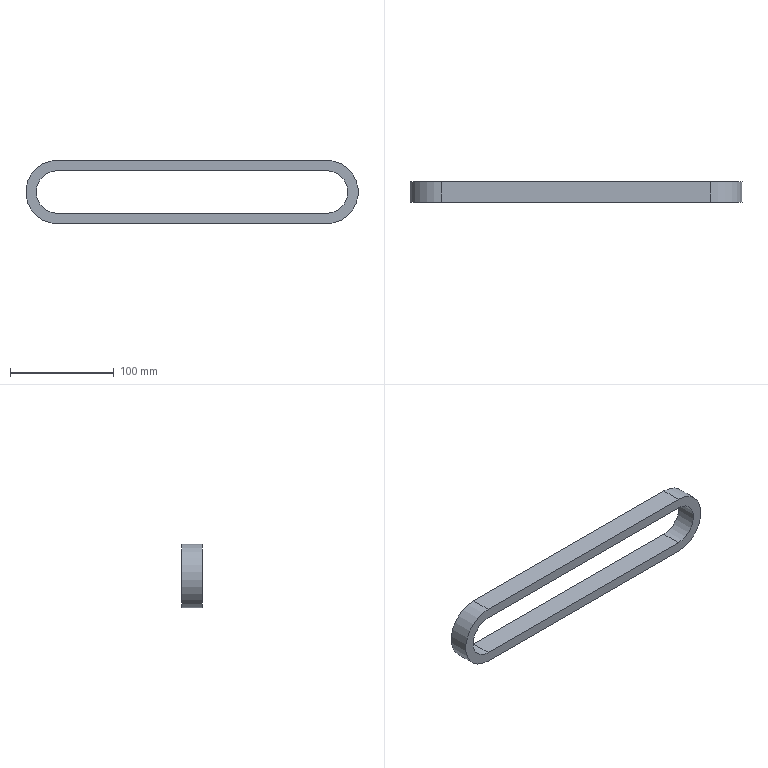Component | NX | MODEL3 | 1 solid | 10 faces | box 320 x 20 x 61 mm | volume 135644 mm3 | plane 6 | cylinder 4 | commonest cylinder face diameters 41 x2 61 x2
STEP:
#1=CARTESIAN_POINT('',(0.,0.,0.));
#2=DIRECTION('',(0.,0.,1.));
#3=DIRECTION('',(1.,0.,0.));
#4=AXIS2_PLACEMENT_3D('',#1,#2,#3);
#5=CARTESIAN_POINT('',(989.5,-5.069,-212.891));
#6=VERTEX_POINT('',#5);
#7=CARTESIAN_POINT('',(730.5,-5.069,-212.891));
#8=VERTEX_POINT('',#7);
#9=CARTESIAN_POINT('',(989.5,-5.069,-212.891));
#10=DIRECTION('',(-1.,0.,0.));
#11=VECTOR('',#10,1.);
#12=LINE('',#9,#11);
#13=CARTESIAN_POINT('',(989.5,-25.069,-212.891));
#14=DIRECTION('',(-0.,0.,-1.));
#15=DIRECTION('',(1.,0.,-0.));
#16=AXIS2_PLACEMENT_3D('',#13,#14,#15);
#17=PLANE('',#16);
#18=CARTESIAN_POINT('',(0.,-20.));
#19=DIRECTION('',(-1.,0.));
#20=VECTOR('',#19,1.);
#21=LINE('',#18,#20);
#22=(GEOMETRIC_REPRESENTATION_CONTEXT(2)PARAMETRIC_REPRESENTATION_CONTEXT()REPRESENTATION_CONTEXT('',''));
#23=DEFINITIONAL_REPRESENTATION('',(#21),#22);
#24=PCURVE('',#17,#23);
#25=CARTESIAN_POINT('',(730.5,-5.069,-192.391));
#26=DIRECTION('',(0.,1.,0.));
#27=DIRECTION('',(0.,0.,-1.));
#28=AXIS2_PLACEMENT_3D('',#25,#26,#27);
#29=PLANE('',#28);
#30=CARTESIAN_POINT('',(20.5,-259.));
#31=DIRECTION('',(-0.,1.));
#32=VECTOR('',#31,1.);
#33=LINE('',#30,#32);
#34=(GEOMETRIC_REPRESENTATION_CONTEXT(2)PARAMETRIC_REPRESENTATION_CONTEXT()REPRESENTATION_CONTEXT('',''));
#35=DEFINITIONAL_REPRESENTATION('',(#33),#34);
#36=PCURVE('',#29,#35);
#37=SURFACE_CURVE('',#12,(#24,#36),.PCURVE_S1.);
#38=EDGE_CURVE('',#6,#8,#37,.T.);
#39=ORIENTED_EDGE('',*,*,#38,.T.);
#40=CARTESIAN_POINT('',(730.5,-25.069,-212.891));
#41=VERTEX_POINT('',#40);
#42=CARTESIAN_POINT('',(730.5,-25.069,-212.891));
#43=DIRECTION('',(0.,1.,0.));
#44=VECTOR('',#43,1.);
#45=LINE('',#42,#44);
#46=CARTESIAN_POINT('',(-259.,0.));
#47=DIRECTION('',(0.,-1.));
#48=VECTOR('',#47,1.);
#49=LINE('',#46,#48);
#50=(GEOMETRIC_REPRESENTATION_CONTEXT(2)PARAMETRIC_REPRESENTATION_CONTEXT()REPRESENTATION_CONTEXT('',''));
#51=DEFINITIONAL_REPRESENTATION('',(#49),#50);
#52=PCURVE('',#17,#51);
#53=CARTESIAN_POINT('',(730.5,-25.069,-192.391));
#54=DIRECTION('',(0.,1.,0.));
#55=DIRECTION('',(0.,0.,-1.));
#56=AXIS2_PLACEMENT_3D('',#53,#54,#55);
#57=CYLINDRICAL_SURFACE('',#56,20.5);
#58=CARTESIAN_POINT('',(0.,0.));
#59=DIRECTION('',(0.,1.));
#60=VECTOR('',#59,1.);
#61=LINE('',#58,#60);
#62=(GEOMETRIC_REPRESENTATION_CONTEXT(2)PARAMETRIC_REPRESENTATION_CONTEXT()REPRESENTATION_CONTEXT('',''));
#63=DEFINITIONAL_REPRESENTATION('',(#61),#62);
#64=PCURVE('',#57,#63);
#65=SURFACE_CURVE('',#45,(#52,#64),.PCURVE_S1.);
#66=EDGE_CURVE('',#41,#8,#65,.T.);
#67=ORIENTED_EDGE('',*,*,#66,.F.);
#68=CARTESIAN_POINT('',(989.5,-25.069,-212.891));
#69=VERTEX_POINT('',#68);
#70=CARTESIAN_POINT('',(989.5,-25.069,-212.891));
#71=DIRECTION('',(-1.,0.,0.));
#72=VECTOR('',#71,1.);
#73=LINE('',#70,#72);
#74=CARTESIAN_POINT('',(0.,0.));
#75=DIRECTION('',(-1.,0.));
#76=VECTOR('',#75,1.);
#77=LINE('',#74,#76);
#78=(GEOMETRIC_REPRESENTATION_CONTEXT(2)PARAMETRIC_REPRESENTATION_CONTEXT()REPRESENTATION_CONTEXT('',''));
#79=DEFINITIONAL_REPRESENTATION('',(#77),#78);
#80=PCURVE('',#17,#79);
#81=CARTESIAN_POINT('',(730.5,-25.069,-192.391));
#82=DIRECTION('',(0.,1.,0.));
#83=DIRECTION('',(0.,0.,-1.));
#84=AXIS2_PLACEMENT_3D('',#81,#82,#83);
#85=PLANE('',#84);
#86=CARTESIAN_POINT('',(20.5,-259.));
#87=DIRECTION('',(-0.,1.));
#88=VECTOR('',#87,1.);
#89=LINE('',#86,#88);
#90=(GEOMETRIC_REPRESENTATION_CONTEXT(2)PARAMETRIC_REPRESENTATION_CONTEXT()REPRESENTATION_CONTEXT('',''));
#91=DEFINITIONAL_REPRESENTATION('',(#89),#90);
#92=PCURVE('',#85,#91);
#93=SURFACE_CURVE('',#73,(#80,#92),.PCURVE_S1.);
#94=EDGE_CURVE('',#69,#41,#93,.T.);
#95=ORIENTED_EDGE('',*,*,#94,.F.);
#96=CARTESIAN_POINT('',(989.5,-25.069,-212.891));
#97=DIRECTION('',(0.,1.,0.));
#98=VECTOR('',#97,1.);
#99=LINE('',#96,#98);
#100=CARTESIAN_POINT('',(0.,0.));
#101=DIRECTION('',(0.,-1.));
#102=VECTOR('',#101,1.);
#103=LINE('',#100,#102);
#104=(GEOMETRIC_REPRESENTATION_CONTEXT(2)PARAMETRIC_REPRESENTATION_CONTEXT()REPRESENTATION_CONTEXT('',''));
#105=DEFINITIONAL_REPRESENTATION('',(#103),#104);
#106=PCURVE('',#17,#105);
#107=CARTESIAN_POINT('',(989.5,-25.069,-192.391));
#108=DIRECTION('',(0.,1.,0.));
#109=DIRECTION('',(0.,0.,-1.));
#110=AXIS2_PLACEMENT_3D('',#107,#108,#109);
#111=CYLINDRICAL_SURFACE('',#110,20.5);
#112=CARTESIAN_POINT('',(6.283,0.));
#113=DIRECTION('',(0.,1.));
#114=VECTOR('',#113,1.);
#115=LINE('',#112,#114);
#116=(GEOMETRIC_REPRESENTATION_CONTEXT(2)PARAMETRIC_REPRESENTATION_CONTEXT()REPRESENTATION_CONTEXT('',''));
#117=DEFINITIONAL_REPRESENTATION('',(#115),#116);
#118=PCURVE('',#111,#117);
#119=SURFACE_CURVE('',#99,(#106,#118),.PCURVE_S1.);
#120=EDGE_CURVE('',#69,#6,#119,.T.);
#121=ORIENTED_EDGE('',*,*,#120,.T.);
#122=EDGE_LOOP('',(#39,#67,#95,#121));
#123=FACE_BOUND('',#122,.T.);
#124=ADVANCED_FACE('',(#123),#17,.F.);
#125=CARTESIAN_POINT('',(989.5,-25.069,-171.891));
#126=VERTEX_POINT('',#125);
#127=CARTESIAN_POINT('',(989.5,-5.069,-171.891));
#128=VERTEX_POINT('',#127);
#129=CARTESIAN_POINT('',(989.5,-25.069,-171.891));
#130=DIRECTION('',(0.,1.,0.));
#131=VECTOR('',#130,1.);
#132=LINE('',#129,#131);
#133=CARTESIAN_POINT('',(3.142,0.));
#134=DIRECTION('',(0.,1.));
#135=VECTOR('',#134,1.);
#136=LINE('',#133,#135);
#137=(GEOMETRIC_REPRESENTATION_CONTEXT(2)PARAMETRIC_REPRESENTATION_CONTEXT()REPRESENTATION_CONTEXT('',''));
#138=DEFINITIONAL_REPRESENTATION('',(#136),#137);
#139=PCURVE('',#111,#138);
#140=CARTESIAN_POINT('',(730.5,-25.069,-171.891));
#141=DIRECTION('',(0.,0.,1.));
#142=DIRECTION('',(-1.,0.,0.));
#143=AXIS2_PLACEMENT_3D('',#140,#141,#142);
#144=PLANE('',#143);
#145=CARTESIAN_POINT('',(-259.,0.));
#146=DIRECTION('',(0.,-1.));
#147=VECTOR('',#146,1.);
#148=LINE('',#145,#147);
#149=(GEOMETRIC_REPRESENTATION_CONTEXT(2)PARAMETRIC_REPRESENTATION_CONTEXT()REPRESENTATION_CONTEXT('',''));
#150=DEFINITIONAL_REPRESENTATION('',(#148),#149);
#151=PCURVE('',#144,#150);
#152=SURFACE_CURVE('',#132,(#139,#151),.PCURVE_S1.);
#153=EDGE_CURVE('',#126,#128,#152,.T.);
#154=ORIENTED_EDGE('',*,*,#153,.F.);
#155=CARTESIAN_POINT('',(989.5,-25.069,-192.391));
#156=DIRECTION('',(0.,1.,0.));
#157=DIRECTION('',(0.,0.,1.));
#158=AXIS2_PLACEMENT_3D('',#155,#156,#157);
#159=CIRCLE('',#158,20.5);
#160=CARTESIAN_POINT('',(3.142,0.));
#161=DIRECTION('',(1.,0.));
#162=VECTOR('',#161,1.);
#163=LINE('',#160,#162);
#164=(GEOMETRIC_REPRESENTATION_CONTEXT(2)PARAMETRIC_REPRESENTATION_CONTEXT()REPRESENTATION_CONTEXT('',''));
#165=DEFINITIONAL_REPRESENTATION('',(#163),#164);
#166=PCURVE('',#111,#165);
#167=CARTESIAN_POINT('',(0.,-259.));
#168=DIRECTION('',(-1.,0.));
#169=AXIS2_PLACEMENT_2D('',#167,#168);
#170=CIRCLE('',#169,20.5);
#171=(GEOMETRIC_REPRESENTATION_CONTEXT(2)PARAMETRIC_REPRESENTATION_CONTEXT()REPRESENTATION_CONTEXT('',''));
#172=DEFINITIONAL_REPRESENTATION('',(#170),#171);
#173=PCURVE('',#85,#172);
#174=SURFACE_CURVE('',#159,(#166,#173),.PCURVE_S1.);
#175=EDGE_CURVE('',#126,#69,#174,.T.);
#176=ORIENTED_EDGE('',*,*,#175,.T.);
#177=ORIENTED_EDGE('',*,*,#120,.T.);
#178=CARTESIAN_POINT('',(989.5,-5.069,-192.391));
#179=DIRECTION('',(0.,1.,0.));
#180=DIRECTION('',(0.,0.,1.));
#181=AXIS2_PLACEMENT_3D('',#178,#179,#180);
#182=CIRCLE('',#181,20.5);
#183=CARTESIAN_POINT('',(3.142,20.));
#184=DIRECTION('',(1.,0.));
#185=VECTOR('',#184,1.);
#186=LINE('',#183,#185);
#187=(GEOMETRIC_REPRESENTATION_CONTEXT(2)PARAMETRIC_REPRESENTATION_CONTEXT()REPRESENTATION_CONTEXT('',''));
#188=DEFINITIONAL_REPRESENTATION('',(#186),#187);
#189=PCURVE('',#111,#188);
#190=CARTESIAN_POINT('',(0.,-259.));
#191=DIRECTION('',(-1.,0.));
#192=AXIS2_PLACEMENT_2D('',#190,#191);
#193=CIRCLE('',#192,20.5);
#194=(GEOMETRIC_REPRESENTATION_CONTEXT(2)PARAMETRIC_REPRESENTATION_CONTEXT()REPRESENTATION_CONTEXT('',''));
#195=DEFINITIONAL_REPRESENTATION('',(#193),#194);
#196=PCURVE('',#29,#195);
#197=SURFACE_CURVE('',#182,(#189,#196),.PCURVE_S1.);
#198=EDGE_CURVE('',#128,#6,#197,.T.);
#199=ORIENTED_EDGE('',*,*,#198,.F.);
#200=EDGE_LOOP('',(#154,#176,#177,#199));
#201=FACE_BOUND('',#200,.F.);
#202=ADVANCED_FACE('',(#201),#111,.F.);
#203=CARTESIAN_POINT('',(730.5,-5.069,-171.891));
#204=VERTEX_POINT('',#203);
#205=CARTESIAN_POINT('',(730.5,-5.069,-171.891));
#206=DIRECTION('',(1.,0.,-0.));
#207=VECTOR('',#206,1.);
#208=LINE('',#205,#207);
#209=CARTESIAN_POINT('',(0.,-20.));
#210=DIRECTION('',(-1.,0.));
#211=VECTOR('',#210,1.);
#212=LINE('',#209,#211);
#213=(GEOMETRIC_REPRESENTATION_CONTEXT(2)PARAMETRIC_REPRESENTATION_CONTEXT()REPRESENTATION_CONTEXT('',''));
#214=DEFINITIONAL_REPRESENTATION('',(#212),#213);
#215=PCURVE('',#144,#214);
#216=CARTESIAN_POINT('',(-20.5,0.));
#217=DIRECTION('',(0.,-1.));
#218=VECTOR('',#217,1.);
#219=LINE('',#216,#218);
#220=(GEOMETRIC_REPRESENTATION_CONTEXT(2)PARAMETRIC_REPRESENTATION_CONTEXT()REPRESENTATION_CONTEXT('',''));
#221=DEFINITIONAL_REPRESENTATION('',(#219),#220);
#222=PCURVE('',#29,#221);
#223=SURFACE_CURVE('',#208,(#215,#222),.PCURVE_S1.);
#224=EDGE_CURVE('',#204,#128,#223,.T.);
#225=ORIENTED_EDGE('',*,*,#224,.T.);
#226=ORIENTED_EDGE('',*,*,#153,.F.);
#227=CARTESIAN_POINT('',(730.5,-25.069,-171.891));
#228=VERTEX_POINT('',#227);
#229=CARTESIAN_POINT('',(730.5,-25.069,-171.891));
#230=DIRECTION('',(1.,0.,-0.));
#231=VECTOR('',#230,1.);
#232=LINE('',#229,#231);
#233=CARTESIAN_POINT('',(0.,0.));
#234=DIRECTION('',(-1.,0.));
#235=VECTOR('',#234,1.);
#236=LINE('',#233,#235);
#237=(GEOMETRIC_REPRESENTATION_CONTEXT(2)PARAMETRIC_REPRESENTATION_CONTEXT()REPRESENTATION_CONTEXT('',''));
#238=DEFINITIONAL_REPRESENTATION('',(#236),#237);
#239=PCURVE('',#144,#238);
#240=CARTESIAN_POINT('',(-20.5,0.));
#241=DIRECTION('',(0.,-1.));
#242=VECTOR('',#241,1.);
#243=LINE('',#240,#242);
#244=(GEOMETRIC_REPRESENTATION_CONTEXT(2)PARAMETRIC_REPRESENTATION_CONTEXT()REPRESENTATION_CONTEXT('',''));
#245=DEFINITIONAL_REPRESENTATION('',(#243),#244);
#246=PCURVE('',#85,#245);
#247=SURFACE_CURVE('',#232,(#239,#246),.PCURVE_S1.);
#248=EDGE_CURVE('',#228,#126,#247,.T.);
#249=ORIENTED_EDGE('',*,*,#248,.F.);
#250=CARTESIAN_POINT('',(730.5,-25.069,-171.891));
#251=DIRECTION('',(0.,1.,0.));
#252=VECTOR('',#251,1.);
#253=LINE('',#250,#252);
#254=CARTESIAN_POINT('',(0.,0.));
#255=DIRECTION('',(0.,-1.));
#256=VECTOR('',#255,1.);
#257=LINE('',#254,#256);
#258=(GEOMETRIC_REPRESENTATION_CONTEXT(2)PARAMETRIC_REPRESENTATION_CONTEXT()REPRESENTATION_CONTEXT('',''));
#259=DEFINITIONAL_REPRESENTATION('',(#257),#258);
#260=PCURVE('',#144,#259);
#261=CARTESIAN_POINT('',(3.142,0.));
#262=DIRECTION('',(0.,1.));
#263=VECTOR('',#262,1.);
#264=LINE('',#261,#263);
#265=(GEOMETRIC_REPRESENTATION_CONTEXT(2)PARAMETRIC_REPRESENTATION_CONTEXT()REPRESENTATION_CONTEXT('',''));
#266=DEFINITIONAL_REPRESENTATION('',(#264),#265);
#267=PCURVE('',#57,#266);
#268=SURFACE_CURVE('',#253,(#260,#267),.PCURVE_S1.);
#269=EDGE_CURVE('',#228,#204,#268,.T.);
#270=ORIENTED_EDGE('',*,*,#269,.T.);
#271=EDGE_LOOP('',(#225,#226,#249,#270));
#272=FACE_BOUND('',#271,.T.);
#273=ADVANCED_FACE('',(#272),#144,.F.);
#274=CARTESIAN_POINT('',(989.5,-5.069,-222.891));
#275=VERTEX_POINT('',#274);
#276=CARTESIAN_POINT('',(730.5,-5.069,-222.891));
#277=VERTEX_POINT('',#276);
#278=CARTESIAN_POINT('',(989.5,-5.069,-222.891));
#279=DIRECTION('',(-1.,0.,0.));
#280=VECTOR('',#279,1.);
#281=LINE('',#278,#280);
#282=CARTESIAN_POINT('',(989.5,-25.069,-222.891));
#283=DIRECTION('',(-0.,0.,-1.));
#284=DIRECTION('',(1.,0.,-0.));
#285=AXIS2_PLACEMENT_3D('',#282,#283,#284);
#286=PLANE('',#285);
#287=CARTESIAN_POINT('',(0.,-20.));
#288=DIRECTION('',(-1.,0.));
#289=VECTOR('',#288,1.);
#290=LINE('',#287,#289);
#291=(GEOMETRIC_REPRESENTATION_CONTEXT(2)PARAMETRIC_REPRESENTATION_CONTEXT()REPRESENTATION_CONTEXT('',''));
#292=DEFINITIONAL_REPRESENTATION('',(#290),#291);
#293=PCURVE('',#286,#292);
#294=CARTESIAN_POINT('',(30.5,-259.));
#295=DIRECTION('',(-0.,1.));
#296=VECTOR('',#295,1.);
#297=LINE('',#294,#296);
#298=(GEOMETRIC_REPRESENTATION_CONTEXT(2)PARAMETRIC_REPRESENTATION_CONTEXT()REPRESENTATION_CONTEXT('',''));
#299=DEFINITIONAL_REPRESENTATION('',(#297),#298);
#300=PCURVE('',#29,#299);
#301=SURFACE_CURVE('',#281,(#293,#300),.PCURVE_S1.);
#302=EDGE_CURVE('',#275,#277,#301,.T.);
#303=ORIENTED_EDGE('',*,*,#302,.F.);
#304=CARTESIAN_POINT('',(989.5,-25.069,-222.891));
#305=VERTEX_POINT('',#304);
#306=CARTESIAN_POINT('',(989.5,-25.069,-222.891));
#307=DIRECTION('',(0.,1.,0.));
#308=VECTOR('',#307,1.);
#309=LINE('',#306,#308);
#310=CARTESIAN_POINT('',(0.,0.));
#311=DIRECTION('',(0.,-1.));
#312=VECTOR('',#311,1.);
#313=LINE('',#310,#312);
#314=(GEOMETRIC_REPRESENTATION_CONTEXT(2)PARAMETRIC_REPRESENTATION_CONTEXT()REPRESENTATION_CONTEXT('',''));
#315=DEFINITIONAL_REPRESENTATION('',(#313),#314);
#316=PCURVE('',#286,#315);
#317=CARTESIAN_POINT('',(989.5,-25.069,-192.391));
#318=DIRECTION('',(0.,1.,0.));
#319=DIRECTION('',(0.,0.,-1.));
#320=AXIS2_PLACEMENT_3D('',#317,#318,#319);
#321=CYLINDRICAL_SURFACE('',#320,30.5);
#322=CARTESIAN_POINT('',(6.283,0.));
#323=DIRECTION('',(0.,1.));
#324=VECTOR('',#323,1.);
#325=LINE('',#322,#324);
#326=(GEOMETRIC_REPRESENTATION_CONTEXT(2)PARAMETRIC_REPRESENTATION_CONTEXT()REPRESENTATION_CONTEXT('',''));
#327=DEFINITIONAL_REPRESENTATION('',(#325),#326);
#328=PCURVE('',#321,#327);
#329=SURFACE_CURVE('',#309,(#316,#328),.PCURVE_S1.);
#330=EDGE_CURVE('',#305,#275,#329,.T.);
#331=ORIENTED_EDGE('',*,*,#330,.F.);
#332=CARTESIAN_POINT('',(730.5,-25.069,-222.891));
#333=VERTEX_POINT('',#332);
#334=CARTESIAN_POINT('',(989.5,-25.069,-222.891));
#335=DIRECTION('',(-1.,0.,0.));
#336=VECTOR('',#335,1.);
#337=LINE('',#334,#336);
#338=CARTESIAN_POINT('',(0.,0.));
#339=DIRECTION('',(-1.,0.));
#340=VECTOR('',#339,1.);
#341=LINE('',#338,#340);
#342=(GEOMETRIC_REPRESENTATION_CONTEXT(2)PARAMETRIC_REPRESENTATION_CONTEXT()REPRESENTATION_CONTEXT('',''));
#343=DEFINITIONAL_REPRESENTATION('',(#341),#342);
#344=PCURVE('',#286,#343);
#345=CARTESIAN_POINT('',(30.5,-259.));
#346=DIRECTION('',(-0.,1.));
#347=VECTOR('',#346,1.);
#348=LINE('',#345,#347);
#349=(GEOMETRIC_REPRESENTATION_CONTEXT(2)PARAMETRIC_REPRESENTATION_CONTEXT()REPRESENTATION_CONTEXT('',''));
#350=DEFINITIONAL_REPRESENTATION('',(#348),#349);
#351=PCURVE('',#85,#350);
#352=SURFACE_CURVE('',#337,(#344,#351),.PCURVE_S1.);
#353=EDGE_CURVE('',#305,#333,#352,.T.);
#354=ORIENTED_EDGE('',*,*,#353,.T.);
#355=CARTESIAN_POINT('',(730.5,-25.069,-222.891));
#356=DIRECTION('',(0.,1.,0.));
#357=VECTOR('',#356,1.);
#358=LINE('',#355,#357);
#359=CARTESIAN_POINT('',(-259.,0.));
#360=DIRECTION('',(0.,-1.));
#361=VECTOR('',#360,1.);
#362=LINE('',#359,#361);
#363=(GEOMETRIC_REPRESENTATION_CONTEXT(2)PARAMETRIC_REPRESENTATION_CONTEXT()REPRESENTATION_CONTEXT('',''));
#364=DEFINITIONAL_REPRESENTATION('',(#362),#363);
#365=PCURVE('',#286,#364);
#366=CARTESIAN_POINT('',(730.5,-25.069,-192.391));
#367=DIRECTION('',(0.,1.,0.));
#368=DIRECTION('',(0.,0.,-1.));
#369=AXIS2_PLACEMENT_3D('',#366,#367,#368);
#370=CYLINDRICAL_SURFACE('',#369,30.5);
#371=CARTESIAN_POINT('',(0.,0.));
#372=DIRECTION('',(0.,1.));
#373=VECTOR('',#372,1.);
#374=LINE('',#371,#373);
#375=(GEOMETRIC_REPRESENTATION_CONTEXT(2)PARAMETRIC_REPRESENTATION_CONTEXT()REPRESENTATION_CONTEXT('',''));
#376=DEFINITIONAL_REPRESENTATION('',(#374),#375);
#377=PCURVE('',#370,#376);
#378=SURFACE_CURVE('',#358,(#365,#377),.PCURVE_S1.);
#379=EDGE_CURVE('',#333,#277,#378,.T.);
#380=ORIENTED_EDGE('',*,*,#379,.T.);
#381=EDGE_LOOP('',(#303,#331,#354,#380));
#382=FACE_BOUND('',#381,.T.);
#383=ADVANCED_FACE('',(#382),#286,.T.);
#384=CARTESIAN_POINT('',(730.5,-5.069,-161.891));
#385=VERTEX_POINT('',#384);
#386=CARTESIAN_POINT('',(730.5,-5.069,-192.391));
#387=DIRECTION('',(0.,1.,0.));
#388=DIRECTION('',(0.,0.,1.));
#389=AXIS2_PLACEMENT_3D('',#386,#387,#388);
#390=CIRCLE('',#389,30.5);
#391=CARTESIAN_POINT('',(-3.142,20.));
#392=DIRECTION('',(1.,0.));
#393=VECTOR('',#392,1.);
#394=LINE('',#391,#393);
#395=(GEOMETRIC_REPRESENTATION_CONTEXT(2)PARAMETRIC_REPRESENTATION_CONTEXT()REPRESENTATION_CONTEXT('',''));
#396=DEFINITIONAL_REPRESENTATION('',(#394),#395);
#397=PCURVE('',#370,#396);
#398=CARTESIAN_POINT('',(0.,0.));
#399=DIRECTION('',(-1.,0.));
#400=AXIS2_PLACEMENT_2D('',#398,#399);
#401=CIRCLE('',#400,30.5);
#402=(GEOMETRIC_REPRESENTATION_CONTEXT(2)PARAMETRIC_REPRESENTATION_CONTEXT()REPRESENTATION_CONTEXT('',''));
#403=DEFINITIONAL_REPRESENTATION('',(#401),#402);
#404=PCURVE('',#29,#403);
#405=SURFACE_CURVE('',#390,(#397,#404),.PCURVE_S1.);
#406=EDGE_CURVE('',#277,#385,#405,.T.);
#407=ORIENTED_EDGE('',*,*,#406,.F.);
#408=ORIENTED_EDGE('',*,*,#379,.F.);
#409=CARTESIAN_POINT('',(730.5,-25.069,-161.891));
#410=VERTEX_POINT('',#409);
#411=CARTESIAN_POINT('',(730.5,-25.069,-192.391));
#412=DIRECTION('',(0.,1.,0.));
#413=DIRECTION('',(0.,0.,1.));
#414=AXIS2_PLACEMENT_3D('',#411,#412,#413);
#415=CIRCLE('',#414,30.5);
#416=CARTESIAN_POINT('',(-3.142,0.));
#417=DIRECTION('',(1.,0.));
#418=VECTOR('',#417,1.);
#419=LINE('',#416,#418);
#420=(GEOMETRIC_REPRESENTATION_CONTEXT(2)PARAMETRIC_REPRESENTATION_CONTEXT()REPRESENTATION_CONTEXT('',''));
#421=DEFINITIONAL_REPRESENTATION('',(#419),#420);
#422=PCURVE('',#370,#421);
#423=CARTESIAN_POINT('',(0.,0.));
#424=DIRECTION('',(-1.,0.));
#425=AXIS2_PLACEMENT_2D('',#423,#424);
#426=CIRCLE('',#425,30.5);
#427=(GEOMETRIC_REPRESENTATION_CONTEXT(2)PARAMETRIC_REPRESENTATION_CONTEXT()REPRESENTATION_CONTEXT('',''));
#428=DEFINITIONAL_REPRESENTATION('',(#426),#427);
#429=PCURVE('',#85,#428);
#430=SURFACE_CURVE('',#415,(#422,#429),.PCURVE_S1.);
#431=EDGE_CURVE('',#333,#410,#430,.T.);
#432=ORIENTED_EDGE('',*,*,#431,.T.);
#433=CARTESIAN_POINT('',(730.5,-25.069,-161.891));
#434=DIRECTION('',(0.,1.,0.));
#435=VECTOR('',#434,1.);
#436=LINE('',#433,#435);
#437=CARTESIAN_POINT('',(3.142,0.));
#438=DIRECTION('',(0.,1.));
#439=VECTOR('',#438,1.);
#440=LINE('',#437,#439);
#441=(GEOMETRIC_REPRESENTATION_CONTEXT(2)PARAMETRIC_REPRESENTATION_CONTEXT()REPRESENTATION_CONTEXT('',''));
#442=DEFINITIONAL_REPRESENTATION('',(#440),#441);
#443=PCURVE('',#370,#442);
#444=CARTESIAN_POINT('',(730.5,-25.069,-161.891));
#445=DIRECTION('',(0.,0.,1.));
#446=DIRECTION('',(-1.,0.,0.));
#447=AXIS2_PLACEMENT_3D('',#444,#445,#446);
#448=PLANE('',#447);
#449=CARTESIAN_POINT('',(0.,0.));
#450=DIRECTION('',(0.,-1.));
#451=VECTOR('',#450,1.);
#452=LINE('',#449,#451);
#453=(GEOMETRIC_REPRESENTATION_CONTEXT(2)PARAMETRIC_REPRESENTATION_CONTEXT()REPRESENTATION_CONTEXT('',''));
#454=DEFINITIONAL_REPRESENTATION('',(#452),#453);
#455=PCURVE('',#448,#454);
#456=SURFACE_CURVE('',#436,(#443,#455),.PCURVE_S1.);
#457=EDGE_CURVE('',#410,#385,#456,.T.);
#458=ORIENTED_EDGE('',*,*,#457,.T.);
#459=EDGE_LOOP('',(#407,#408,#432,#458));
#460=FACE_BOUND('',#459,.T.);
#461=ADVANCED_FACE('',(#460),#370,.T.);
#462=CARTESIAN_POINT('',(989.5,-5.069,-161.891));
#463=VERTEX_POINT('',#462);
#464=CARTESIAN_POINT('',(730.5,-5.069,-161.891));
#465=DIRECTION('',(1.,0.,-0.));
#466=VECTOR('',#465,1.);
#467=LINE('',#464,#466);
#468=CARTESIAN_POINT('',(0.,-20.));
#469=DIRECTION('',(-1.,0.));
#470=VECTOR('',#469,1.);
#471=LINE('',#468,#470);
#472=(GEOMETRIC_REPRESENTATION_CONTEXT(2)PARAMETRIC_REPRESENTATION_CONTEXT()REPRESENTATION_CONTEXT('',''));
#473=DEFINITIONAL_REPRESENTATION('',(#471),#472);
#474=PCURVE('',#448,#473);
#475=CARTESIAN_POINT('',(-30.5,0.));
#476=DIRECTION('',(0.,-1.));
#477=VECTOR('',#476,1.);
#478=LINE('',#475,#477);
#479=(GEOMETRIC_REPRESENTATION_CONTEXT(2)PARAMETRIC_REPRESENTATION_CONTEXT()REPRESENTATION_CONTEXT('',''));
#480=DEFINITIONAL_REPRESENTATION('',(#478),#479);
#481=PCURVE('',#29,#480);
#482=SURFACE_CURVE('',#467,(#474,#481),.PCURVE_S1.);
#483=EDGE_CURVE('',#385,#463,#482,.T.);
#484=ORIENTED_EDGE('',*,*,#483,.F.);
#485=ORIENTED_EDGE('',*,*,#457,.F.);
#486=CARTESIAN_POINT('',(989.5,-25.069,-161.891));
#487=VERTEX_POINT('',#486);
#488=CARTESIAN_POINT('',(730.5,-25.069,-161.891));
#489=DIRECTION('',(1.,0.,-0.));
#490=VECTOR('',#489,1.);
#491=LINE('',#488,#490);
#492=CARTESIAN_POINT('',(0.,0.));
#493=DIRECTION('',(-1.,0.));
#494=VECTOR('',#493,1.);
#495=LINE('',#492,#494);
#496=(GEOMETRIC_REPRESENTATION_CONTEXT(2)PARAMETRIC_REPRESENTATION_CONTEXT()REPRESENTATION_CONTEXT('',''));
#497=DEFINITIONAL_REPRESENTATION('',(#495),#496);
#498=PCURVE('',#448,#497);
#499=CARTESIAN_POINT('',(-30.5,0.));
#500=DIRECTION('',(0.,-1.));
#501=VECTOR('',#500,1.);
#502=LINE('',#499,#501);
#503=(GEOMETRIC_REPRESENTATION_CONTEXT(2)PARAMETRIC_REPRESENTATION_CONTEXT()REPRESENTATION_CONTEXT('',''));
#504=DEFINITIONAL_REPRESENTATION('',(#502),#503);
#505=PCURVE('',#85,#504);
#506=SURFACE_CURVE('',#491,(#498,#505),.PCURVE_S1.);
#507=EDGE_CURVE('',#410,#487,#506,.T.);
#508=ORIENTED_EDGE('',*,*,#507,.T.);
#509=CARTESIAN_POINT('',(989.5,-25.069,-161.891));
#510=DIRECTION('',(0.,1.,0.));
#511=VECTOR('',#510,1.);
#512=LINE('',#509,#511);
#513=CARTESIAN_POINT('',(-259.,0.));
#514=DIRECTION('',(0.,-1.));
#515=VECTOR('',#514,1.);
#516=LINE('',#513,#515);
#517=(GEOMETRIC_REPRESENTATION_CONTEXT(2)PARAMETRIC_REPRESENTATION_CONTEXT()REPRESENTATION_CONTEXT('',''));
#518=DEFINITIONAL_REPRESENTATION('',(#516),#517);
#519=PCURVE('',#448,#518);
#520=CARTESIAN_POINT('',(3.142,0.));
#521=DIRECTION('',(0.,1.));
#522=VECTOR('',#521,1.);
#523=LINE('',#520,#522);
#524=(GEOMETRIC_REPRESENTATION_CONTEXT(2)PARAMETRIC_REPRESENTATION_CONTEXT()REPRESENTATION_CONTEXT('',''));
#525=DEFINITIONAL_REPRESENTATION('',(#523),#524);
#526=PCURVE('',#321,#525);
#527=SURFACE_CURVE('',#512,(#519,#526),.PCURVE_S1.);
#528=EDGE_CURVE('',#487,#463,#527,.T.);
#529=ORIENTED_EDGE('',*,*,#528,.T.);
#530=EDGE_LOOP('',(#484,#485,#508,#529));
#531=FACE_BOUND('',#530,.T.);
#532=ADVANCED_FACE('',(#531),#448,.T.);
#533=CARTESIAN_POINT('',(989.5,-5.069,-192.391));
#534=DIRECTION('',(0.,1.,0.));
#535=DIRECTION('',(0.,0.,1.));
#536=AXIS2_PLACEMENT_3D('',#533,#534,#535);
#537=CIRCLE('',#536,30.5);
#538=CARTESIAN_POINT('',(3.142,20.));
#539=DIRECTION('',(1.,0.));
#540=VECTOR('',#539,1.);
#541=LINE('',#538,#540);
#542=(GEOMETRIC_REPRESENTATION_CONTEXT(2)PARAMETRIC_REPRESENTATION_CONTEXT()REPRESENTATION_CONTEXT('',''));
#543=DEFINITIONAL_REPRESENTATION('',(#541),#542);
#544=PCURVE('',#321,#543);
#545=CARTESIAN_POINT('',(0.,-259.));
#546=DIRECTION('',(-1.,0.));
#547=AXIS2_PLACEMENT_2D('',#545,#546);
#548=CIRCLE('',#547,30.5);
#549=(GEOMETRIC_REPRESENTATION_CONTEXT(2)PARAMETRIC_REPRESENTATION_CONTEXT()REPRESENTATION_CONTEXT('',''));
#550=DEFINITIONAL_REPRESENTATION('',(#548),#549);
#551=PCURVE('',#29,#550);
#552=SURFACE_CURVE('',#537,(#544,#551),.PCURVE_S1.);
#553=EDGE_CURVE('',#463,#275,#552,.T.);
#554=ORIENTED_EDGE('',*,*,#553,.F.);
#555=ORIENTED_EDGE('',*,*,#528,.F.);
#556=CARTESIAN_POINT('',(989.5,-25.069,-192.391));
#557=DIRECTION('',(0.,1.,0.));
#558=DIRECTION('',(0.,0.,1.));
#559=AXIS2_PLACEMENT_3D('',#556,#557,#558);
#560=CIRCLE('',#559,30.5);
#561=CARTESIAN_POINT('',(3.142,0.));
#562=DIRECTION('',(1.,0.));
#563=VECTOR('',#562,1.);
#564=LINE('',#561,#563);
#565=(GEOMETRIC_REPRESENTATION_CONTEXT(2)PARAMETRIC_REPRESENTATION_CONTEXT()REPRESENTATION_CONTEXT('',''));
#566=DEFINITIONAL_REPRESENTATION('',(#564),#565);
#567=PCURVE('',#321,#566);
#568=CARTESIAN_POINT('',(0.,-259.));
#569=DIRECTION('',(-1.,0.));
#570=AXIS2_PLACEMENT_2D('',#568,#569);
#571=CIRCLE('',#570,30.5);
#572=(GEOMETRIC_REPRESENTATION_CONTEXT(2)PARAMETRIC_REPRESENTATION_CONTEXT()REPRESENTATION_CONTEXT('',''));
#573=DEFINITIONAL_REPRESENTATION('',(#571),#572);
#574=PCURVE('',#85,#573);
#575=SURFACE_CURVE('',#560,(#567,#574),.PCURVE_S1.);
#576=EDGE_CURVE('',#487,#305,#575,.T.);
#577=ORIENTED_EDGE('',*,*,#576,.T.);
#578=ORIENTED_EDGE('',*,*,#330,.T.);
#579=EDGE_LOOP('',(#554,#555,#577,#578));
#580=FACE_BOUND('',#579,.T.);
#581=ADVANCED_FACE('',(#580),#321,.T.);
#582=ORIENTED_EDGE('',*,*,#66,.F.);
#583=CARTESIAN_POINT('',(730.5,-25.069,-192.391));
#584=DIRECTION('',(0.,1.,0.));
#585=DIRECTION('',(0.,0.,1.));
#586=AXIS2_PLACEMENT_3D('',#583,#584,#585);
#587=CIRCLE('',#586,20.5);
#588=CARTESIAN_POINT('',(-3.142,0.));
#589=DIRECTION('',(1.,0.));
#590=VECTOR('',#589,1.);
#591=LINE('',#588,#590);
#592=(GEOMETRIC_REPRESENTATION_CONTEXT(2)PARAMETRIC_REPRESENTATION_CONTEXT()REPRESENTATION_CONTEXT('',''));
#593=DEFINITIONAL_REPRESENTATION('',(#591),#592);
#594=PCURVE('',#57,#593);
#595=CARTESIAN_POINT('',(0.,0.));
#596=DIRECTION('',(-1.,0.));
#597=AXIS2_PLACEMENT_2D('',#595,#596);
#598=CIRCLE('',#597,20.5);
#599=(GEOMETRIC_REPRESENTATION_CONTEXT(2)PARAMETRIC_REPRESENTATION_CONTEXT()REPRESENTATION_CONTEXT('',''));
#600=DEFINITIONAL_REPRESENTATION('',(#598),#599);
#601=PCURVE('',#85,#600);
#602=SURFACE_CURVE('',#587,(#594,#601),.PCURVE_S1.);
#603=EDGE_CURVE('',#41,#228,#602,.T.);
#604=ORIENTED_EDGE('',*,*,#603,.T.);
#605=ORIENTED_EDGE('',*,*,#269,.T.);
#606=CARTESIAN_POINT('',(730.5,-5.069,-192.391));
#607=DIRECTION('',(0.,1.,0.));
#608=DIRECTION('',(0.,0.,1.));
#609=AXIS2_PLACEMENT_3D('',#606,#607,#608);
#610=CIRCLE('',#609,20.5);
#611=CARTESIAN_POINT('',(-3.142,20.));
#612=DIRECTION('',(1.,0.));
#613=VECTOR('',#612,1.);
#614=LINE('',#611,#613);
#615=(GEOMETRIC_REPRESENTATION_CONTEXT(2)PARAMETRIC_REPRESENTATION_CONTEXT()REPRESENTATION_CONTEXT('',''));
#616=DEFINITIONAL_REPRESENTATION('',(#614),#615);
#617=PCURVE('',#57,#616);
#618=CARTESIAN_POINT('',(0.,0.));
#619=DIRECTION('',(-1.,0.));
#620=AXIS2_PLACEMENT_2D('',#618,#619);
#621=CIRCLE('',#620,20.5);
#622=(GEOMETRIC_REPRESENTATION_CONTEXT(2)PARAMETRIC_REPRESENTATION_CONTEXT()REPRESENTATION_CONTEXT('',''));
#623=DEFINITIONAL_REPRESENTATION('',(#621),#622);
#624=PCURVE('',#29,#623);
#625=SURFACE_CURVE('',#610,(#617,#624),.PCURVE_S1.);
#626=EDGE_CURVE('',#8,#204,#625,.T.);
#627=ORIENTED_EDGE('',*,*,#626,.F.);
#628=EDGE_LOOP('',(#582,#604,#605,#627));
#629=FACE_BOUND('',#628,.F.);
#630=ADVANCED_FACE('',(#629),#57,.F.);
#631=ORIENTED_EDGE('',*,*,#353,.F.);
#632=ORIENTED_EDGE('',*,*,#576,.F.);
#633=ORIENTED_EDGE('',*,*,#507,.F.);
#634=ORIENTED_EDGE('',*,*,#431,.F.);
#635=EDGE_LOOP('',(#631,#632,#633,#634));
#636=FACE_BOUND('',#635,.T.);
#637=ORIENTED_EDGE('',*,*,#94,.T.);
#638=ORIENTED_EDGE('',*,*,#603,.T.);
#639=ORIENTED_EDGE('',*,*,#248,.T.);
#640=ORIENTED_EDGE('',*,*,#175,.T.);
#641=EDGE_LOOP('',(#637,#638,#639,#640));
#642=FACE_BOUND('',#641,.T.);
#643=ADVANCED_FACE('',(#636,#642),#85,.F.);
#644=ORIENTED_EDGE('',*,*,#302,.T.);
#645=ORIENTED_EDGE('',*,*,#406,.T.);
#646=ORIENTED_EDGE('',*,*,#483,.T.);
#647=ORIENTED_EDGE('',*,*,#553,.T.);
#648=EDGE_LOOP('',(#644,#645,#646,#647));
#649=FACE_BOUND('',#648,.T.);
#650=ORIENTED_EDGE('',*,*,#38,.F.);
#651=ORIENTED_EDGE('',*,*,#198,.F.);
#652=ORIENTED_EDGE('',*,*,#224,.F.);
#653=ORIENTED_EDGE('',*,*,#626,.F.);
#654=EDGE_LOOP('',(#650,#651,#652,#653));
#655=FACE_BOUND('',#654,.T.);
#656=ADVANCED_FACE('',(#649,#655),#29,.T.);
#657=CLOSED_SHELL('',(#124,#202,#273,#383,#461,#532,#581,#630,#643,#656));
#658=MANIFOLD_SOLID_BREP('',#657);
#659=(LENGTH_UNIT()NAMED_UNIT(*)SI_UNIT(.MILLI.,.METRE.));
#660=UNCERTAINTY_MEASURE_WITH_UNIT(LENGTH_MEASURE(0.0000001),#659,'','');
#661=(NAMED_UNIT(*)PLANE_ANGLE_UNIT()SI_UNIT($,.RADIAN.));
#662=(NAMED_UNIT(*)SI_UNIT($,.STERADIAN.)SOLID_ANGLE_UNIT());
#663=(GEOMETRIC_REPRESENTATION_CONTEXT(3)GLOBAL_UNCERTAINTY_ASSIGNED_CONTEXT((#660))GLOBAL_UNIT_ASSIGNED_CONTEXT((#659,#661,#662))REPRESENTATION_CONTEXT('',''));
#664=ADVANCED_BREP_SHAPE_REPRESENTATION('',(#4,#658),#663);